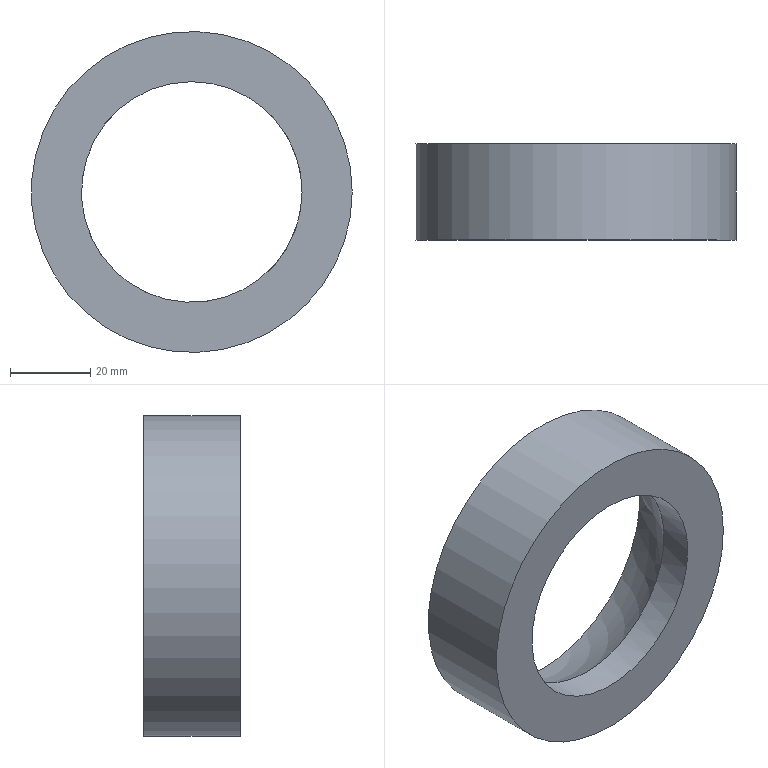Component | NX | FIXED_PAD | 1 solid | 5 faces | box 80 x 24 x 80 mm | volume 51033 mm3 | cylinder 2 | plane 2 | sphere 1 | commonest cylinder face diameters 80 x1 55 x1
STEP:
#1=CARTESIAN_POINT('',(0.,0.,0.));
#2=DIRECTION('',(0.,0.,1.));
#3=DIRECTION('',(1.,0.,0.));
#4=AXIS2_PLACEMENT_3D('',#1,#2,#3);
#5=CARTESIAN_POINT('',(223.939,-30.,60.622));
#6=VERTEX_POINT('',#5);
#7=CARTESIAN_POINT('',(183.939,-30.,60.622));
#8=DIRECTION('',(0.,-1.,0.));
#9=DIRECTION('',(1.,0.,0.));
#10=AXIS2_PLACEMENT_3D('',#7,#8,#9);
#11=CIRCLE('',#10,40.);
#12=CARTESIAN_POINT('',(183.939,-30.,60.622));
#13=DIRECTION('',(0.,1.,0.));
#14=DIRECTION('',(0.,0.,1.));
#15=AXIS2_PLACEMENT_3D('',#12,#13,#14);
#16=CYLINDRICAL_SURFACE('',#15,40.);
#17=CARTESIAN_POINT('',(7.854,0.));
#18=DIRECTION('',(-1.,0.));
#19=VECTOR('',#18,1.);
#20=LINE('',#17,#19);
#21=(GEOMETRIC_REPRESENTATION_CONTEXT(2)PARAMETRIC_REPRESENTATION_CONTEXT()REPRESENTATION_CONTEXT('',''));
#22=DEFINITIONAL_REPRESENTATION('',(#20),#21);
#23=PCURVE('',#16,#22);
#24=CARTESIAN_POINT('',(183.939,-30.,60.622));
#25=DIRECTION('',(0.,-1.,0.));
#26=DIRECTION('',(0.,0.,-1.));
#27=AXIS2_PLACEMENT_3D('',#24,#25,#26);
#28=PLANE('',#27);
#29=CARTESIAN_POINT('',(0.,0.));
#30=DIRECTION('',(0.,1.));
#31=AXIS2_PLACEMENT_2D('',#29,#30);
#32=CIRCLE('',#31,40.);
#33=(GEOMETRIC_REPRESENTATION_CONTEXT(2)PARAMETRIC_REPRESENTATION_CONTEXT()REPRESENTATION_CONTEXT('',''));
#34=DEFINITIONAL_REPRESENTATION('',(#32),#33);
#35=PCURVE('',#28,#34);
#36=SURFACE_CURVE('',#11,(#23,#35),.PCURVE_S1.);
#37=EDGE_CURVE('',#6,#6,#36,.T.);
#38=ORIENTED_EDGE('',*,*,#37,.F.);
#39=CARTESIAN_POINT('',(223.939,-6.,60.622));
#40=VERTEX_POINT('',#39);
#41=CARTESIAN_POINT('',(223.939,-30.,60.622));
#42=CARTESIAN_POINT('',(223.939,-6.,60.622));
#43=B_SPLINE_CURVE_WITH_KNOTS('',1,(#41,#42),.UNSPECIFIED.,.F.,.F.,(2,2),(0.,24.),.PIECEWISE_BEZIER_KNOTS.);
#44=CARTESIAN_POINT('',(7.854,0.));
#45=DIRECTION('',(0.,1.));
#46=VECTOR('',#45,1.);
#47=LINE('',#44,#46);
#48=(GEOMETRIC_REPRESENTATION_CONTEXT(2)PARAMETRIC_REPRESENTATION_CONTEXT()REPRESENTATION_CONTEXT('',''));
#49=DEFINITIONAL_REPRESENTATION('',(#47),#48);
#50=PCURVE('',#16,#49);
#51=CARTESIAN_POINT('',(1.571,0.));
#52=DIRECTION('',(0.,1.));
#53=VECTOR('',#52,1.);
#54=LINE('',#51,#53);
#55=(GEOMETRIC_REPRESENTATION_CONTEXT(2)PARAMETRIC_REPRESENTATION_CONTEXT()REPRESENTATION_CONTEXT('',''));
#56=DEFINITIONAL_REPRESENTATION('',(#54),#55);
#57=PCURVE('',#16,#56);
#58=SEAM_CURVE('',#43,(#50,#57),.PCURVE_S1.);
#59=EDGE_CURVE('',#6,#40,#58,.T.);
#60=ORIENTED_EDGE('',*,*,#59,.T.);
#61=CARTESIAN_POINT('',(183.939,-6.,60.622));
#62=DIRECTION('',(0.,-1.,0.));
#63=DIRECTION('',(1.,0.,0.));
#64=AXIS2_PLACEMENT_3D('',#61,#62,#63);
#65=CIRCLE('',#64,40.);
#66=CARTESIAN_POINT('',(7.854,24.));
#67=DIRECTION('',(-1.,0.));
#68=VECTOR('',#67,1.);
#69=LINE('',#66,#68);
#70=(GEOMETRIC_REPRESENTATION_CONTEXT(2)PARAMETRIC_REPRESENTATION_CONTEXT()REPRESENTATION_CONTEXT('',''));
#71=DEFINITIONAL_REPRESENTATION('',(#69),#70);
#72=PCURVE('',#16,#71);
#73=CARTESIAN_POINT('',(183.939,-6.,60.622));
#74=DIRECTION('',(0.,-1.,0.));
#75=DIRECTION('',(0.,0.,-1.));
#76=AXIS2_PLACEMENT_3D('',#73,#74,#75);
#77=PLANE('',#76);
#78=CARTESIAN_POINT('',(0.,0.));
#79=DIRECTION('',(0.,1.));
#80=AXIS2_PLACEMENT_2D('',#78,#79);
#81=CIRCLE('',#80,40.);
#82=(GEOMETRIC_REPRESENTATION_CONTEXT(2)PARAMETRIC_REPRESENTATION_CONTEXT()REPRESENTATION_CONTEXT('',''));
#83=DEFINITIONAL_REPRESENTATION('',(#81),#82);
#84=PCURVE('',#77,#83);
#85=SURFACE_CURVE('',#65,(#72,#84),.PCURVE_S1.);
#86=EDGE_CURVE('',#40,#40,#85,.T.);
#87=ORIENTED_EDGE('',*,*,#86,.T.);
#88=ORIENTED_EDGE('',*,*,#59,.F.);
#89=EDGE_LOOP('',(#38,#60,#87,#88));
#90=FACE_BOUND('',#89,.T.);
#91=ADVANCED_FACE('',(#90),#16,.T.);
#92=CARTESIAN_POINT('',(183.939,-21.651,88.122));
#93=VERTEX_POINT('',#92);
#94=CARTESIAN_POINT('',(183.939,-21.651,60.622));
#95=DIRECTION('',(0.,-1.,0.));
#96=DIRECTION('',(0.,0.,1.));
#97=AXIS2_PLACEMENT_3D('',#94,#95,#96);
#98=CIRCLE('',#97,27.5);
#99=CARTESIAN_POINT('',(183.939,-30.,60.622));
#100=DIRECTION('',(0.,1.,0.));
#101=DIRECTION('',(0.,0.,1.));
#102=AXIS2_PLACEMENT_3D('',#99,#100,#101);
#103=CYLINDRICAL_SURFACE('',#102,27.5);
#104=CARTESIAN_POINT('',(6.283,8.349));
#105=DIRECTION('',(-1.,0.));
#106=VECTOR('',#105,1.);
#107=LINE('',#104,#106);
#108=(GEOMETRIC_REPRESENTATION_CONTEXT(2)PARAMETRIC_REPRESENTATION_CONTEXT()REPRESENTATION_CONTEXT('',''));
#109=DEFINITIONAL_REPRESENTATION('',(#107),#108);
#110=PCURVE('',#103,#109);
#111=CARTESIAN_POINT('',(183.939,-0.,60.622));
#112=DIRECTION('',(0.,0.,1.));
#113=DIRECTION('',(1.,0.,0.));
#114=AXIS2_PLACEMENT_3D('',#111,#112,#113);
#115=SPHERICAL_SURFACE('',#114,35.);
#116=CARTESIAN_POINT('',(4.712,0.9038));
#117=CARTESIAN_POINT('',(4.585,0.9044));
#118=CARTESIAN_POINT('',(4.355,0.8677));
#119=CARTESIAN_POINT('',(4.093,0.7301));
#120=CARTESIAN_POINT('',(3.936,0.5446));
#121=CARTESIAN_POINT('',(3.847,0.3344));
#122=CARTESIAN_POINT('',(3.807,0.1126));
#123=CARTESIAN_POINT('',(3.807,-0.1126));
#124=CARTESIAN_POINT('',(3.847,-0.3344));
#125=CARTESIAN_POINT('',(3.936,-0.5446));
#126=CARTESIAN_POINT('',(4.094,-0.7301));
#127=CARTESIAN_POINT('',(4.351,-0.868));
#128=CARTESIAN_POINT('',(4.712,-0.9218));
#129=CARTESIAN_POINT('',(5.073,-0.868));
#130=CARTESIAN_POINT('',(5.331,-0.7301));
#131=CARTESIAN_POINT('',(5.489,-0.5446));
#132=CARTESIAN_POINT('',(5.578,-0.3344));
#133=CARTESIAN_POINT('',(5.618,-0.1126));
#134=CARTESIAN_POINT('',(5.618,0.1126));
#135=CARTESIAN_POINT('',(5.578,0.3344));
#136=CARTESIAN_POINT('',(5.489,0.5446));
#137=CARTESIAN_POINT('',(5.332,0.7301));
#138=CARTESIAN_POINT('',(5.07,0.8677));
#139=CARTESIAN_POINT('',(4.84,0.9044));
#140=CARTESIAN_POINT('',(4.712,0.9038));
#141=B_SPLINE_CURVE_WITH_KNOTS('',3,(#116,#117,#118,#119,#120,#121,#122,#123,#124,#125,#126,#127,#128,#129,#130,#131,#132,#133,#134,#135,#136,#137,#138,#139,#140),.UNSPECIFIED.,.T.,.F.,(4,1,1,1,1,1,1,1,1,1,1,1,1,1,1,1,1,1,1,1,1,1,4),(0.,0.2856,0.5712,0.8568,1.142,1.428,1.714,1.999,2.285,2.57,2.856,3.142,3.427,3.713,3.998,4.284,4.57,4.855,5.141,5.426,5.712,5.998,6.283),.QUASI_UNIFORM_KNOTS.);
#142=(GEOMETRIC_REPRESENTATION_CONTEXT(2)PARAMETRIC_REPRESENTATION_CONTEXT()REPRESENTATION_CONTEXT('',''));
#143=DEFINITIONAL_REPRESENTATION('',(#141),#142);
#144=PCURVE('',#115,#143);
#145=SURFACE_CURVE('',#98,(#110,#144),.PCURVE_S1.);
#146=EDGE_CURVE('',#93,#93,#145,.T.);
#147=ORIENTED_EDGE('',*,*,#146,.T.);
#148=CARTESIAN_POINT('',(183.939,-30.,88.122));
#149=VERTEX_POINT('',#148);
#150=CARTESIAN_POINT('',(183.939,-30.,88.122));
#151=CARTESIAN_POINT('',(183.939,-21.651,88.122));
#152=B_SPLINE_CURVE_WITH_KNOTS('',1,(#150,#151),.UNSPECIFIED.,.F.,.F.,(2,2),(0.,8.349),.PIECEWISE_BEZIER_KNOTS.);
#153=CARTESIAN_POINT('',(0.,0.));
#154=DIRECTION('',(0.,1.));
#155=VECTOR('',#154,1.);
#156=LINE('',#153,#155);
#157=(GEOMETRIC_REPRESENTATION_CONTEXT(2)PARAMETRIC_REPRESENTATION_CONTEXT()REPRESENTATION_CONTEXT('',''));
#158=DEFINITIONAL_REPRESENTATION('',(#156),#157);
#159=PCURVE('',#103,#158);
#160=CARTESIAN_POINT('',(6.283,0.));
#161=DIRECTION('',(0.,1.));
#162=VECTOR('',#161,1.);
#163=LINE('',#160,#162);
#164=(GEOMETRIC_REPRESENTATION_CONTEXT(2)PARAMETRIC_REPRESENTATION_CONTEXT()REPRESENTATION_CONTEXT('',''));
#165=DEFINITIONAL_REPRESENTATION('',(#163),#164);
#166=PCURVE('',#103,#165);
#167=SEAM_CURVE('',#152,(#159,#166),.PCURVE_S1.);
#168=EDGE_CURVE('',#149,#93,#167,.T.);
#169=ORIENTED_EDGE('',*,*,#168,.F.);
#170=CARTESIAN_POINT('',(211.439,-30.,60.622));
#171=VERTEX_POINT('',#170);
#172=CARTESIAN_POINT('',(183.939,-30.,60.622));
#173=DIRECTION('',(0.,-1.,0.));
#174=DIRECTION('',(1.,0.,0.));
#175=AXIS2_PLACEMENT_3D('',#172,#173,#174);
#176=CIRCLE('',#175,27.5);
#177=CARTESIAN_POINT('',(1.571,0.));
#178=DIRECTION('',(-1.,0.));
#179=VECTOR('',#178,1.);
#180=LINE('',#177,#179);
#181=(GEOMETRIC_REPRESENTATION_CONTEXT(2)PARAMETRIC_REPRESENTATION_CONTEXT()REPRESENTATION_CONTEXT('',''));
#182=DEFINITIONAL_REPRESENTATION('',(#180),#181);
#183=PCURVE('',#103,#182);
#184=CARTESIAN_POINT('',(0.,0.));
#185=DIRECTION('',(0.,1.));
#186=AXIS2_PLACEMENT_2D('',#184,#185);
#187=CIRCLE('',#186,27.5);
#188=(GEOMETRIC_REPRESENTATION_CONTEXT(2)PARAMETRIC_REPRESENTATION_CONTEXT()REPRESENTATION_CONTEXT('',''));
#189=DEFINITIONAL_REPRESENTATION('',(#187),#188);
#190=PCURVE('',#28,#189);
#191=SURFACE_CURVE('',#176,(#183,#190),.PCURVE_S1.);
#192=EDGE_CURVE('',#171,#149,#191,.T.);
#193=ORIENTED_EDGE('',*,*,#192,.F.);
#194=CARTESIAN_POINT('',(183.939,-30.,60.622));
#195=DIRECTION('',(0.,-1.,0.));
#196=DIRECTION('',(1.,0.,0.));
#197=AXIS2_PLACEMENT_3D('',#194,#195,#196);
#198=CIRCLE('',#197,27.5);
#199=CARTESIAN_POINT('',(7.854,0.));
#200=DIRECTION('',(-1.,0.));
#201=VECTOR('',#200,1.);
#202=LINE('',#199,#201);
#203=(GEOMETRIC_REPRESENTATION_CONTEXT(2)PARAMETRIC_REPRESENTATION_CONTEXT()REPRESENTATION_CONTEXT('',''));
#204=DEFINITIONAL_REPRESENTATION('',(#202),#203);
#205=PCURVE('',#103,#204);
#206=CARTESIAN_POINT('',(0.,0.));
#207=DIRECTION('',(0.,1.));
#208=AXIS2_PLACEMENT_2D('',#206,#207);
#209=CIRCLE('',#208,27.5);
#210=(GEOMETRIC_REPRESENTATION_CONTEXT(2)PARAMETRIC_REPRESENTATION_CONTEXT()REPRESENTATION_CONTEXT('',''));
#211=DEFINITIONAL_REPRESENTATION('',(#209),#210);
#212=PCURVE('',#28,#211);
#213=SURFACE_CURVE('',#198,(#205,#212),.PCURVE_S1.);
#214=EDGE_CURVE('',#149,#171,#213,.T.);
#215=ORIENTED_EDGE('',*,*,#214,.F.);
#216=ORIENTED_EDGE('',*,*,#168,.T.);
#217=EDGE_LOOP('',(#147,#169,#193,#215,#216));
#218=FACE_BOUND('',#217,.F.);
#219=ADVANCED_FACE('',(#218),#103,.F.);
#220=ORIENTED_EDGE('',*,*,#37,.T.);
#221=EDGE_LOOP('',(#220));
#222=FACE_BOUND('',#221,.T.);
#223=ORIENTED_EDGE('',*,*,#192,.F.);
#224=ORIENTED_EDGE('',*,*,#214,.F.);
#225=EDGE_LOOP('',(#223,#224));
#226=FACE_BOUND('',#225,.T.);
#227=ADVANCED_FACE('',(#222,#226),#28,.T.);
#228=CARTESIAN_POINT('',(183.939,-6.,26.14));
#229=VERTEX_POINT('',#228);
#230=CARTESIAN_POINT('',(183.939,-6.,60.622));
#231=DIRECTION('',(0.,-1.,0.));
#232=DIRECTION('',(0.,0.,-1.));
#233=AXIS2_PLACEMENT_3D('',#230,#231,#232);
#234=CIRCLE('',#233,34.482);
#235=CARTESIAN_POINT('',(0.,0.));
#236=DIRECTION('',(1.,0.));
#237=AXIS2_PLACEMENT_2D('',#235,#236);
#238=CIRCLE('',#237,34.482);
#239=(GEOMETRIC_REPRESENTATION_CONTEXT(2)PARAMETRIC_REPRESENTATION_CONTEXT()REPRESENTATION_CONTEXT('',''));
#240=DEFINITIONAL_REPRESENTATION('',(#238),#239);
#241=PCURVE('',#77,#240);
#242=CARTESIAN_POINT('',(4.712,-1.399));
#243=CARTESIAN_POINT('',(5.25,-1.372));
#244=CARTESIAN_POINT('',(5.866,-1.256));
#245=CARTESIAN_POINT('',(5.974,-0.9757));
#246=CARTESIAN_POINT('',(6.068,-0.7025));
#247=CARTESIAN_POINT('',(6.096,-0.4216));
#248=CARTESIAN_POINT('',(6.112,-0.1408));
#249=CARTESIAN_POINT('',(6.112,0.1407));
#250=CARTESIAN_POINT('',(6.095,0.4219));
#251=CARTESIAN_POINT('',(6.072,0.7016));
#252=CARTESIAN_POINT('',(5.958,0.979));
#253=CARTESIAN_POINT('',(5.927,1.244));
#254=CARTESIAN_POINT('',(4.712,1.476));
#255=CARTESIAN_POINT('',(3.497,1.244));
#256=CARTESIAN_POINT('',(3.467,0.979));
#257=CARTESIAN_POINT('',(3.353,0.7016));
#258=CARTESIAN_POINT('',(3.33,0.4219));
#259=CARTESIAN_POINT('',(3.313,0.1407));
#260=CARTESIAN_POINT('',(3.313,-0.1408));
#261=CARTESIAN_POINT('',(3.328,-0.4216));
#262=CARTESIAN_POINT('',(3.357,-0.7025));
#263=CARTESIAN_POINT('',(3.45,-0.9757));
#264=CARTESIAN_POINT('',(3.559,-1.256));
#265=CARTESIAN_POINT('',(4.175,-1.372));
#266=CARTESIAN_POINT('',(4.712,-1.399));
#267=B_SPLINE_CURVE_WITH_KNOTS('',3,(#242,#243,#244,#245,#246,#247,#248,#249,#250,#251,#252,#253,#254,#255,#256,#257,#258,#259,#260,#261,#262,#263,#264,#265,#266),.UNSPECIFIED.,.T.,.F.,(4,1,1,1,1,1,1,1,1,1,1,1,1,1,1,1,1,1,1,1,1,1,4),(0.,0.2856,0.5712,0.8568,1.142,1.428,1.714,1.999,2.285,2.57,2.856,3.142,3.427,3.713,3.998,4.284,4.57,4.855,5.141,5.426,5.712,5.998,6.283),.QUASI_UNIFORM_KNOTS.);
#268=(GEOMETRIC_REPRESENTATION_CONTEXT(2)PARAMETRIC_REPRESENTATION_CONTEXT()REPRESENTATION_CONTEXT('',''));
#269=DEFINITIONAL_REPRESENTATION('',(#267),#268);
#270=PCURVE('',#115,#269);
#271=SURFACE_CURVE('',#234,(#241,#270),.PCURVE_S1.);
#272=EDGE_CURVE('',#229,#229,#271,.T.);
#273=ORIENTED_EDGE('',*,*,#272,.T.);
#274=EDGE_LOOP('',(#273));
#275=FACE_BOUND('',#274,.T.);
#276=ORIENTED_EDGE('',*,*,#86,.F.);
#277=EDGE_LOOP('',(#276));
#278=FACE_BOUND('',#277,.T.);
#279=ADVANCED_FACE('',(#275,#278),#77,.F.);
#280=ORIENTED_EDGE('',*,*,#146,.F.);
#281=EDGE_LOOP('',(#280));
#282=FACE_BOUND('',#281,.F.);
#283=ORIENTED_EDGE('',*,*,#272,.T.);
#284=EDGE_LOOP('',(#283));
#285=FACE_BOUND('',#284,.F.);
#286=ADVANCED_FACE('',(#282,#285),#115,.F.);
#287=CLOSED_SHELL('',(#91,#219,#227,#279,#286));
#288=MANIFOLD_SOLID_BREP('',#287);
#289=(LENGTH_UNIT()NAMED_UNIT(*)SI_UNIT(.MILLI.,.METRE.));
#290=UNCERTAINTY_MEASURE_WITH_UNIT(LENGTH_MEASURE(0.000005),#289,'','');
#291=(NAMED_UNIT(*)PLANE_ANGLE_UNIT()SI_UNIT($,.RADIAN.));
#292=(NAMED_UNIT(*)SI_UNIT($,.STERADIAN.)SOLID_ANGLE_UNIT());
#293=(GEOMETRIC_REPRESENTATION_CONTEXT(3)GLOBAL_UNCERTAINTY_ASSIGNED_CONTEXT((#290))GLOBAL_UNIT_ASSIGNED_CONTEXT((#289,#291,#292))REPRESENTATION_CONTEXT('',''));
#294=ADVANCED_BREP_SHAPE_REPRESENTATION('',(#4,#288),#293);